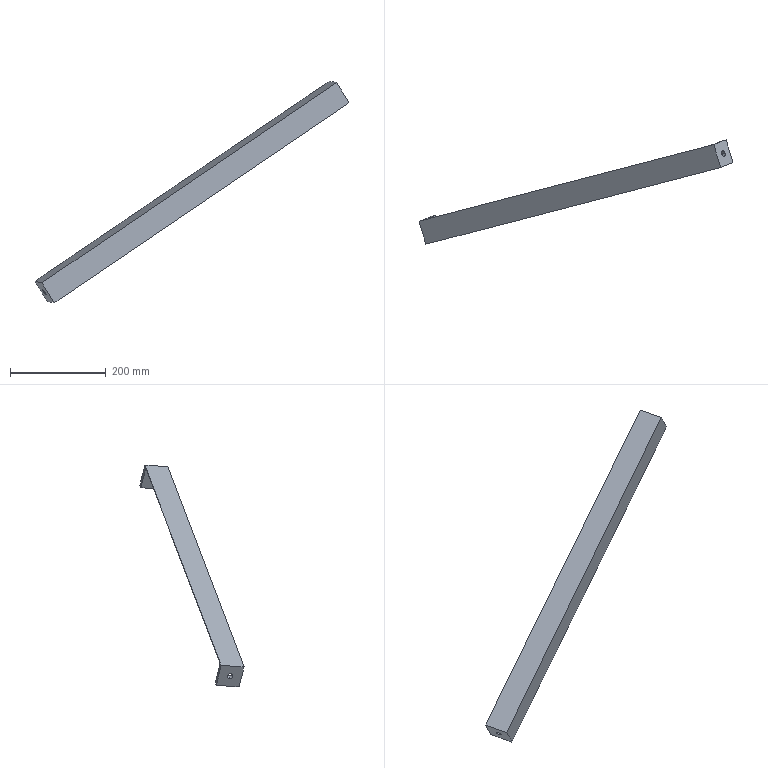Component | SolidWorks | CrusherFrameSpacer-1 | 1 solid | 19 faces | box 654.75 x 217.27 x 462.26 mm | volume 399079 mm3 | plane 12 | cylinder 7 | commonest cylinder face diameters 12 x4 10 x2 14 x1
build123d program:
from build123d import *

# Parameters (mm, degrees)
EXTRUDE2_DEPTH     = 760
SKETCH3_W          = 50
SKETCH3_H          = 50
EXTRUDE3_DEPTH     = 10
SKETCH4_W          = 50
SKETCH4_H          = 50
EXTRUDE4_DEPTH     = 10
SKETCH5_R          = 6
CUT_EXTRUDE1_DEPTH = 763.129


with BuildPart() as part:
    # Sketch2 → Extrude2 (new body)
    with BuildSketch(Plane.XY):
        with BuildLine():
            Line((-22.775, 0), (-22.775, 50))
            ThreePointArc((-22.775, 50), (-19.239, 48.536), (-17.775, 45))
            Line((-17.775, 45), (-17.775, 12))
            ThreePointArc((-17.775, 12), (-15.725, 7.05), (-10.775, 5))
            Line((-10.775, 5), (22.225, 5))
            ThreePointArc((22.225, 5), (25.761, 3.536), (27.225, 0))
            Line((27.225, 0), (-22.775, 0))
        make_face()
    extrude(amount=EXTRUDE2_DEPTH)

    # Sketch3 → Extrude3 (add)
    with BuildSketch(Plane.XY.offset(760)):
        with Locations((2.225, 25)):
            Rectangle(SKETCH3_W, SKETCH3_H)
    extrude(amount=-EXTRUDE3_DEPTH)

    # Sketch4 → Extrude4 (add)
    with BuildSketch(Plane(origin=(0, 0, 0), x_dir=(-1, 0, 0), z_dir=(0, 0, -1))):
        with Locations((-2.225, 25)):
            Rectangle(SKETCH4_W, SKETCH4_H)
    extrude(amount=-EXTRUDE4_DEPTH)

    # Sketch5 → Cut-Extrude1 (cut, through all)
    with BuildSketch(Plane(origin=(0, 0, 0), x_dir=(-1, 0, 0), z_dir=(0, 0, -1))):
        with Locations((-2.225, 25)):
            Circle(SKETCH5_R)
    extrude(amount=-CUT_EXTRUDE1_DEPTH, mode=Mode.SUBTRACT)


solid = part.part

# Placed as in the assembly
solid = solid.moved(Location((-230.699, -92.36, -620.774), (-20.862, 53.982, 29.322)))
STEP:
#1=CARTESIAN_POINT('',(15.001,3.637,-8.21));
#2=VERTEX_POINT('',#1);
#3=CARTESIAN_POINT('',(14.759,3.54,-7.816));
#4=VERTEX_POINT('',#3);
#5=CARTESIAN_POINT('',(14.88,3.589,-8.013));
#6=DIRECTION('',(-0.8088,-0.2094,-0.5495));
#7=DIRECTION('',(-0.5127,-0.2065,0.8334));
#8=AXIS2_PLACEMENT_3D('',#5,#6,#7);
#9=CIRCLE('',#8,0.2362);
#10=EDGE_CURVE('',#2,#4,#9,.T.);
#11=ORIENTED_EDGE('',*,*,#10,.F.);
#12=CARTESIAN_POINT('',(14.683,3.555,-8.426));
#13=VERTEX_POINT('',#12);
#14=CARTESIAN_POINT('',(15.001,3.637,-8.21));
#15=DIRECTION('',(-0.8088,-0.2094,-0.5495));
#16=VECTOR('',#15,39.37);
#17=LINE('',#14,#16);
#18=EDGE_CURVE('',#2,#13,#17,.T.);
#19=ORIENTED_EDGE('',*,*,#18,.T.);
#20=CARTESIAN_POINT('',(14.441,3.457,-8.032));
#21=VERTEX_POINT('',#20);
#22=CARTESIAN_POINT('',(14.562,3.506,-8.229));
#23=DIRECTION('',(0.8088,0.2094,0.5495));
#24=DIRECTION('',(0.5127,0.2065,-0.8334));
#25=AXIS2_PLACEMENT_3D('',#22,#23,#24);
#26=CIRCLE('',#25,0.2362);
#27=EDGE_CURVE('',#21,#13,#26,.T.);
#28=ORIENTED_EDGE('',*,*,#27,.F.);
#29=CARTESIAN_POINT('',(14.759,3.54,-7.816));
#30=DIRECTION('',(-0.8088,-0.2094,-0.5495));
#31=VECTOR('',#30,39.37);
#32=LINE('',#29,#31);
#33=EDGE_CURVE('',#4,#21,#32,.T.);
#34=ORIENTED_EDGE('',*,*,#33,.F.);
#35=EDGE_LOOP('',(#11,#19,#28,#34));
#36=FACE_OUTER_BOUND('',#35,.T.);
#37=CARTESIAN_POINT('',(14.88,3.589,-8.013));
#38=DIRECTION('',(-0.8088,-0.2094,-0.5495));
#39=DIRECTION('',(-0.5127,-0.2065,0.8334));
#40=AXIS2_PLACEMENT_3D('',#37,#38,#39);
#41=CYLINDRICAL_SURFACE('',#40,0.2362);
#42=ADVANCED_FACE('',(#36),#41,.F.);
#43=CARTESIAN_POINT('',(-8.882,-2.546,-24.435));
#44=VERTEX_POINT('',#43);
#45=CARTESIAN_POINT('',(-9.124,-2.644,-24.041));
#46=VERTEX_POINT('',#45);
#47=CARTESIAN_POINT('',(-9.003,-2.595,-24.238));
#48=DIRECTION('',(-0.8088,-0.2094,-0.5495));
#49=DIRECTION('',(-0.5127,-0.2065,0.8334));
#50=AXIS2_PLACEMENT_3D('',#47,#48,#49);
#51=CIRCLE('',#50,0.2362);
#52=EDGE_CURVE('',#44,#46,#51,.T.);
#53=ORIENTED_EDGE('',*,*,#52,.F.);
#54=CARTESIAN_POINT('',(-9.2,-2.629,-24.651));
#55=VERTEX_POINT('',#54);
#56=CARTESIAN_POINT('',(15.001,3.637,-8.21));
#57=DIRECTION('',(-0.8088,-0.2094,-0.5495));
#58=VECTOR('',#57,39.37);
#59=LINE('',#56,#58);
#60=EDGE_CURVE('',#44,#55,#59,.T.);
#61=ORIENTED_EDGE('',*,*,#60,.T.);
#62=CARTESIAN_POINT('',(-9.442,-2.726,-24.257));
#63=VERTEX_POINT('',#62);
#64=CARTESIAN_POINT('',(-9.321,-2.677,-24.454));
#65=DIRECTION('',(-0.8088,-0.2094,-0.5495));
#66=DIRECTION('',(-0.5127,-0.2065,0.8334));
#67=AXIS2_PLACEMENT_3D('',#64,#65,#66);
#68=CIRCLE('',#67,0.2362);
#69=EDGE_CURVE('',#55,#63,#68,.T.);
#70=ORIENTED_EDGE('',*,*,#69,.T.);
#71=CARTESIAN_POINT('',(14.759,3.54,-7.816));
#72=DIRECTION('',(-0.8088,-0.2094,-0.5495));
#73=VECTOR('',#72,39.37);
#74=LINE('',#71,#73);
#75=EDGE_CURVE('',#46,#63,#74,.T.);
#76=ORIENTED_EDGE('',*,*,#75,.F.);
#77=EDGE_LOOP('',(#53,#61,#70,#76));
#78=FACE_OUTER_BOUND('',#77,.T.);
#79=CARTESIAN_POINT('',(14.88,3.589,-8.013));
#80=DIRECTION('',(-0.8088,-0.2094,-0.5495));
#81=DIRECTION('',(-0.5127,-0.2065,0.8334));
#82=AXIS2_PLACEMENT_3D('',#79,#80,#81);
#83=CYLINDRICAL_SURFACE('',#82,0.2362);
#84=ADVANCED_FACE('',(#78),#83,.F.);
#85=CARTESIAN_POINT('',(-8.372,-3.185,-24.941));
#86=VERTEX_POINT('',#85);
#87=CARTESIAN_POINT('',(-8.215,-3.332,-25.117));
#88=VERTEX_POINT('',#87);
#89=CARTESIAN_POINT('',(-8.316,-3.373,-24.953));
#90=DIRECTION('',(-0.8088,-0.2094,-0.5495));
#91=DIRECTION('',(-0.5127,-0.2065,0.8334));
#92=AXIS2_PLACEMENT_3D('',#89,#90,#91);
#93=CIRCLE('',#92,0.1969);
#94=EDGE_CURVE('',#86,#88,#93,.T.);
#95=ORIENTED_EDGE('',*,*,#94,.F.);
#96=CARTESIAN_POINT('',(15.192,2.916,-8.932));
#97=VERTEX_POINT('',#96);
#98=CARTESIAN_POINT('',(15.511,2.999,-8.716));
#99=DIRECTION('',(-0.8088,-0.2094,-0.5495));
#100=VECTOR('',#99,39.37);
#101=LINE('',#98,#100);
#102=EDGE_CURVE('',#97,#86,#101,.T.);
#103=ORIENTED_EDGE('',*,*,#102,.F.);
#104=CARTESIAN_POINT('',(15.35,2.769,-9.108));
#105=VERTEX_POINT('',#104);
#106=CARTESIAN_POINT('',(15.249,2.728,-8.944));
#107=DIRECTION('',(0.8088,0.2094,0.5495));
#108=DIRECTION('',(0.5127,0.2065,-0.8334));
#109=AXIS2_PLACEMENT_3D('',#106,#107,#108);
#110=CIRCLE('',#109,0.1969);
#111=EDGE_CURVE('',#105,#97,#110,.T.);
#112=ORIENTED_EDGE('',*,*,#111,.F.);
#113=CARTESIAN_POINT('',(15.668,2.851,-8.892));
#114=DIRECTION('',(-0.8088,-0.2094,-0.5495));
#115=VECTOR('',#114,39.37);
#116=LINE('',#113,#115);
#117=EDGE_CURVE('',#105,#88,#116,.T.);
#118=ORIENTED_EDGE('',*,*,#117,.T.);
#119=EDGE_LOOP('',(#95,#103,#112,#118));
#120=FACE_OUTER_BOUND('',#119,.T.);
#121=CARTESIAN_POINT('',(15.567,2.81,-8.728));
#122=DIRECTION('',(-0.8088,-0.2094,-0.5495));
#123=DIRECTION('',(-0.5127,-0.2065,0.8334));
#124=AXIS2_PLACEMENT_3D('',#121,#122,#123);
#125=CYLINDRICAL_SURFACE('',#124,0.1969);
#126=ADVANCED_FACE('',(#120),#125,.T.);
#127=CARTESIAN_POINT('',(-9.038,-3.453,-23.858));
#128=VERTEX_POINT('',#127);
#129=CARTESIAN_POINT('',(-8.372,-3.185,-24.941));
#130=DIRECTION('',(0.5127,0.2065,-0.8334));
#131=VECTOR('',#130,39.37);
#132=LINE('',#129,#131);
#133=EDGE_CURVE('',#128,#86,#132,.T.);
#134=ORIENTED_EDGE('',*,*,#133,.F.);
#135=CARTESIAN_POINT('',(14.526,2.648,-7.85));
#136=VERTEX_POINT('',#135);
#137=CARTESIAN_POINT('',(14.845,2.73,-7.633));
#138=DIRECTION('',(-0.8088,-0.2094,-0.5495));
#139=VECTOR('',#138,39.37);
#140=LINE('',#137,#139);
#141=EDGE_CURVE('',#136,#128,#140,.T.);
#142=ORIENTED_EDGE('',*,*,#141,.F.);
#143=CARTESIAN_POINT('',(15.192,2.916,-8.932));
#144=DIRECTION('',(-0.5127,-0.2065,0.8334));
#145=VECTOR('',#144,39.37);
#146=LINE('',#143,#145);
#147=EDGE_CURVE('',#97,#136,#146,.T.);
#148=ORIENTED_EDGE('',*,*,#147,.F.);
#149=ORIENTED_EDGE('',*,*,#102,.T.);
#150=EDGE_LOOP('',(#134,#142,#148,#149));
#151=FACE_OUTER_BOUND('',#150,.T.);
#152=CARTESIAN_POINT('',(15.511,2.999,-8.716));
#153=DIRECTION('',(0.288,-0.9558,-0.05964));
#154=DIRECTION('',(0.5127,0.2065,-0.8334));
#155=AXIS2_PLACEMENT_3D('',#152,#153,#154);
#156=PLANE('',#155);
#157=ADVANCED_FACE('',(#151),#156,.F.);
#158=CARTESIAN_POINT('',(-9.259,-3.247,-23.612));
#159=VERTEX_POINT('',#158);
#160=CARTESIAN_POINT('',(-9.118,-3.19,-23.842));
#161=DIRECTION('',(0.8088,0.2094,0.5495));
#162=DIRECTION('',(-0.5127,-0.2065,0.8334));
#163=AXIS2_PLACEMENT_3D('',#160,#161,#162);
#164=CIRCLE('',#163,0.2756);
#165=EDGE_CURVE('',#159,#128,#164,.T.);
#166=ORIENTED_EDGE('',*,*,#165,.F.);
#167=CARTESIAN_POINT('',(14.305,2.854,-7.604));
#168=VERTEX_POINT('',#167);
#169=CARTESIAN_POINT('',(14.624,2.937,-7.387));
#170=DIRECTION('',(-0.8088,-0.2094,-0.5495));
#171=VECTOR('',#170,39.37);
#172=LINE('',#169,#171);
#173=EDGE_CURVE('',#168,#159,#172,.T.);
#174=ORIENTED_EDGE('',*,*,#173,.F.);
#175=CARTESIAN_POINT('',(14.447,2.911,-7.833));
#176=DIRECTION('',(-0.8088,-0.2094,-0.5495));
#177=DIRECTION('',(0.5127,0.2065,-0.8334));
#178=AXIS2_PLACEMENT_3D('',#175,#176,#177);
#179=CIRCLE('',#178,0.2756);
#180=EDGE_CURVE('',#136,#168,#179,.T.);
#181=ORIENTED_EDGE('',*,*,#180,.F.);
#182=ORIENTED_EDGE('',*,*,#141,.T.);
#183=EDGE_LOOP('',(#166,#174,#181,#182));
#184=FACE_OUTER_BOUND('',#183,.T.);
#185=CARTESIAN_POINT('',(14.765,2.994,-7.617));
#186=DIRECTION('',(-0.8088,-0.2094,-0.5495));
#187=DIRECTION('',(-0.5127,-0.2065,0.8334));
#188=AXIS2_PLACEMENT_3D('',#185,#186,#187);
#189=CYLINDRICAL_SURFACE('',#188,0.2756);
#190=ADVANCED_FACE('',(#184),#189,.F.);
#191=CARTESIAN_POINT('',(-9.633,-2.005,-23.535));
#192=VERTEX_POINT('',#191);
#193=CARTESIAN_POINT('',(-9.633,-2.005,-23.535));
#194=DIRECTION('',(0.288,-0.9558,-0.05964));
#195=VECTOR('',#194,39.37);
#196=LINE('',#193,#195);
#197=EDGE_CURVE('',#192,#159,#196,.T.);
#198=ORIENTED_EDGE('',*,*,#197,.F.);
#199=CARTESIAN_POINT('',(13.931,4.096,-7.526));
#200=VERTEX_POINT('',#199);
#201=CARTESIAN_POINT('',(14.25,4.179,-7.31));
#202=DIRECTION('',(-0.8088,-0.2094,-0.5495));
#203=VECTOR('',#202,39.37);
#204=LINE('',#201,#203);
#205=EDGE_CURVE('',#200,#192,#204,.T.);
#206=ORIENTED_EDGE('',*,*,#205,.F.);
#207=CARTESIAN_POINT('',(13.931,4.096,-7.526));
#208=DIRECTION('',(-0.288,0.9558,0.05964));
#209=VECTOR('',#208,39.37);
#210=LINE('',#207,#209);
#211=EDGE_CURVE('',#168,#200,#210,.T.);
#212=ORIENTED_EDGE('',*,*,#211,.F.);
#213=ORIENTED_EDGE('',*,*,#173,.T.);
#214=EDGE_LOOP('',(#198,#206,#212,#213));
#215=FACE_OUTER_BOUND('',#214,.T.);
#216=CARTESIAN_POINT('',(14.25,4.179,-7.31));
#217=DIRECTION('',(-0.5127,-0.2065,0.8334));
#218=DIRECTION('',(0.288,-0.9558,-0.05964));
#219=AXIS2_PLACEMENT_3D('',#216,#217,#218);
#220=PLANE('',#219);
#221=ADVANCED_FACE('',(#215),#220,.F.);
#222=CARTESIAN_POINT('',(-9.791,-1.857,-23.359));
#223=VERTEX_POINT('',#222);
#224=CARTESIAN_POINT('',(-9.734,-2.046,-23.371));
#225=DIRECTION('',(-0.8088,-0.2094,-0.5495));
#226=DIRECTION('',(-0.5127,-0.2065,0.8334));
#227=AXIS2_PLACEMENT_3D('',#224,#225,#226);
#228=CIRCLE('',#227,0.1969);
#229=EDGE_CURVE('',#223,#192,#228,.T.);
#230=ORIENTED_EDGE('',*,*,#229,.F.);
#231=CARTESIAN_POINT('',(13.774,4.244,-7.35));
#232=VERTEX_POINT('',#231);
#233=CARTESIAN_POINT('',(14.092,4.326,-7.134));
#234=DIRECTION('',(-0.8088,-0.2094,-0.5495));
#235=VECTOR('',#234,39.37);
#236=LINE('',#233,#235);
#237=EDGE_CURVE('',#232,#223,#236,.T.);
#238=ORIENTED_EDGE('',*,*,#237,.F.);
#239=CARTESIAN_POINT('',(13.83,4.055,-7.362));
#240=DIRECTION('',(0.8088,0.2094,0.5495));
#241=DIRECTION('',(0.5127,0.2065,-0.8334));
#242=AXIS2_PLACEMENT_3D('',#239,#240,#241);
#243=CIRCLE('',#242,0.1969);
#244=EDGE_CURVE('',#200,#232,#243,.T.);
#245=ORIENTED_EDGE('',*,*,#244,.F.);
#246=ORIENTED_EDGE('',*,*,#205,.T.);
#247=EDGE_LOOP('',(#230,#238,#245,#246));
#248=FACE_OUTER_BOUND('',#247,.T.);
#249=CARTESIAN_POINT('',(14.149,4.138,-7.146));
#250=DIRECTION('',(-0.8088,-0.2094,-0.5495));
#251=DIRECTION('',(-0.5127,-0.2065,0.8334));
#252=AXIS2_PLACEMENT_3D('',#249,#250,#251);
#253=CYLINDRICAL_SURFACE('',#252,0.1969);
#254=ADVANCED_FACE('',(#248),#253,.T.);
#255=CARTESIAN_POINT('',(-8.533,-3.415,-25.333));
#256=VERTEX_POINT('',#255);
#257=CARTESIAN_POINT('',(-8.215,-3.332,-25.117));
#258=DIRECTION('',(-0.8088,-0.2094,-0.5495));
#259=VECTOR('',#258,39.37);
#260=LINE('',#257,#259);
#261=EDGE_CURVE('',#88,#256,#260,.T.);
#262=ORIENTED_EDGE('',*,*,#261,.F.);
#263=ORIENTED_EDGE('',*,*,#117,.F.);
#264=CARTESIAN_POINT('',(15.668,2.851,-8.892));
#265=VERTEX_POINT('',#264);
#266=CARTESIAN_POINT('',(15.668,2.851,-8.892));
#267=DIRECTION('',(-0.8088,-0.2094,-0.5495));
#268=VECTOR('',#267,39.37);
#269=LINE('',#266,#268);
#270=EDGE_CURVE('',#265,#105,#269,.T.);
#271=ORIENTED_EDGE('',*,*,#270,.F.);
#272=CARTESIAN_POINT('',(14.659,2.445,-7.251));
#273=VERTEX_POINT('',#272);
#274=CARTESIAN_POINT('',(14.659,2.445,-7.251));
#275=DIRECTION('',(0.5127,0.2065,-0.8334));
#276=VECTOR('',#275,39.37);
#277=LINE('',#274,#276);
#278=EDGE_CURVE('',#273,#265,#277,.T.);
#279=ORIENTED_EDGE('',*,*,#278,.F.);
#280=CARTESIAN_POINT('',(-9.542,-3.821,-23.693));
#281=VERTEX_POINT('',#280);
#282=CARTESIAN_POINT('',(14.659,2.445,-7.251));
#283=DIRECTION('',(-0.8088,-0.2094,-0.5495));
#284=VECTOR('',#283,39.37);
#285=LINE('',#282,#284);
#286=EDGE_CURVE('',#273,#281,#285,.T.);
#287=ORIENTED_EDGE('',*,*,#286,.T.);
#288=CARTESIAN_POINT('',(-9.542,-3.821,-23.693));
#289=DIRECTION('',(0.5127,0.2065,-0.8334));
#290=VECTOR('',#289,39.37);
#291=LINE('',#288,#290);
#292=EDGE_CURVE('',#281,#256,#291,.T.);
#293=ORIENTED_EDGE('',*,*,#292,.T.);
#294=EDGE_LOOP('',(#262,#263,#271,#279,#287,#293));
#295=FACE_OUTER_BOUND('',#294,.T.);
#296=CARTESIAN_POINT('',(14.659,2.445,-7.251));
#297=DIRECTION('',(-0.288,0.9558,0.05964));
#298=DIRECTION('',(-0.5127,-0.2065,0.8334));
#299=AXIS2_PLACEMENT_3D('',#296,#297,#298);
#300=PLANE('',#299);
#301=ADVANCED_FACE('',(#295),#300,.F.);
#302=CARTESIAN_POINT('',(-10.109,-1.94,-23.575));
#303=VERTEX_POINT('',#302);
#304=CARTESIAN_POINT('',(-9.542,-3.821,-23.693));
#305=DIRECTION('',(0.288,-0.9558,-0.05964));
#306=VECTOR('',#305,39.37);
#307=LINE('',#304,#306);
#308=EDGE_CURVE('',#303,#281,#307,.T.);
#309=ORIENTED_EDGE('',*,*,#308,.T.);
#310=ORIENTED_EDGE('',*,*,#286,.F.);
#311=CARTESIAN_POINT('',(14.092,4.326,-7.134));
#312=VERTEX_POINT('',#311);
#313=CARTESIAN_POINT('',(14.659,2.445,-7.251));
#314=DIRECTION('',(0.288,-0.9558,-0.05964));
#315=VECTOR('',#314,39.37);
#316=LINE('',#313,#315);
#317=EDGE_CURVE('',#312,#273,#316,.T.);
#318=ORIENTED_EDGE('',*,*,#317,.F.);
#319=CARTESIAN_POINT('',(14.092,4.326,-7.134));
#320=DIRECTION('',(-0.8088,-0.2094,-0.5495));
#321=VECTOR('',#320,39.37);
#322=LINE('',#319,#321);
#323=EDGE_CURVE('',#312,#232,#322,.T.);
#324=ORIENTED_EDGE('',*,*,#323,.T.);
#325=ORIENTED_EDGE('',*,*,#237,.T.);
#326=CARTESIAN_POINT('',(-9.791,-1.857,-23.359));
#327=DIRECTION('',(-0.8088,-0.2094,-0.5495));
#328=VECTOR('',#327,39.37);
#329=LINE('',#326,#328);
#330=EDGE_CURVE('',#223,#303,#329,.T.);
#331=ORIENTED_EDGE('',*,*,#330,.T.);
#332=EDGE_LOOP('',(#309,#310,#318,#324,#325,#331));
#333=FACE_OUTER_BOUND('',#332,.T.);
#334=CARTESIAN_POINT('',(14.659,2.445,-7.251));
#335=DIRECTION('',(0.5127,0.2065,-0.8334));
#336=DIRECTION('',(-0.288,0.9558,0.05964));
#337=AXIS2_PLACEMENT_3D('',#334,#335,#336);
#338=PLANE('',#337);
#339=ADVANCED_FACE('',(#333),#338,.F.);
#340=CARTESIAN_POINT('',(14.88,3.589,-8.013));
#341=DIRECTION('',(-0.8088,-0.2094,-0.5495));
#342=DIRECTION('',(-0.5127,-0.2065,0.8334));
#343=AXIS2_PLACEMENT_3D('',#340,#341,#342);
#344=CIRCLE('',#343,0.2362);
#345=EDGE_CURVE('',#4,#2,#344,.T.);
#346=ORIENTED_EDGE('',*,*,#345,.T.);
#347=ORIENTED_EDGE('',*,*,#10,.T.);
#348=EDGE_LOOP('',(#346,#347));
#349=FACE_BOUND('',#348,.T.);
#350=ORIENTED_EDGE('',*,*,#278,.T.);
#351=CARTESIAN_POINT('',(15.101,4.733,-8.775));
#352=VERTEX_POINT('',#351);
#353=CARTESIAN_POINT('',(15.668,2.851,-8.892));
#354=DIRECTION('',(-0.288,0.9558,0.05964));
#355=VECTOR('',#354,39.37);
#356=LINE('',#353,#355);
#357=EDGE_CURVE('',#265,#352,#356,.T.);
#358=ORIENTED_EDGE('',*,*,#357,.T.);
#359=CARTESIAN_POINT('',(15.101,4.733,-8.775));
#360=DIRECTION('',(-0.5127,-0.2065,0.8334));
#361=VECTOR('',#360,39.37);
#362=LINE('',#359,#361);
#363=EDGE_CURVE('',#352,#312,#362,.T.);
#364=ORIENTED_EDGE('',*,*,#363,.T.);
#365=ORIENTED_EDGE('',*,*,#317,.T.);
#366=EDGE_LOOP('',(#350,#358,#364,#365));
#367=FACE_OUTER_BOUND('',#366,.T.);
#368=CARTESIAN_POINT('',(15.567,2.81,-8.728));
#369=DIRECTION('',(-0.8088,-0.2094,-0.5495));
#370=DIRECTION('',(-0.5127,-0.2065,0.8334));
#371=AXIS2_PLACEMENT_3D('',#368,#369,#370);
#372=PLANE('',#371);
#373=ADVANCED_FACE('',(#349,#367),#372,.F.);
#374=CARTESIAN_POINT('',(-9.321,-2.677,-24.454));
#375=DIRECTION('',(-0.8088,-0.2094,-0.5495));
#376=DIRECTION('',(-0.5127,-0.2065,0.8334));
#377=AXIS2_PLACEMENT_3D('',#374,#375,#376);
#378=CIRCLE('',#377,0.2362);
#379=EDGE_CURVE('',#63,#55,#378,.T.);
#380=ORIENTED_EDGE('',*,*,#379,.F.);
#381=ORIENTED_EDGE('',*,*,#69,.F.);
#382=EDGE_LOOP('',(#380,#381));
#383=FACE_BOUND('',#382,.T.);
#384=ORIENTED_EDGE('',*,*,#292,.F.);
#385=ORIENTED_EDGE('',*,*,#308,.F.);
#386=CARTESIAN_POINT('',(-9.1,-1.533,-25.216));
#387=VERTEX_POINT('',#386);
#388=CARTESIAN_POINT('',(-9.1,-1.533,-25.216));
#389=DIRECTION('',(0.5127,0.2065,-0.8334));
#390=VECTOR('',#389,39.37);
#391=LINE('',#388,#390);
#392=EDGE_CURVE('',#303,#387,#391,.T.);
#393=ORIENTED_EDGE('',*,*,#392,.T.);
#394=CARTESIAN_POINT('',(-9.1,-1.533,-25.216));
#395=DIRECTION('',(0.288,-0.9558,-0.05964));
#396=VECTOR('',#395,39.37);
#397=LINE('',#394,#396);
#398=EDGE_CURVE('',#387,#256,#397,.T.);
#399=ORIENTED_EDGE('',*,*,#398,.T.);
#400=EDGE_LOOP('',(#384,#385,#393,#399));
#401=FACE_OUTER_BOUND('',#400,.T.);
#402=CARTESIAN_POINT('',(-8.634,-3.456,-25.169));
#403=DIRECTION('',(-0.8088,-0.2094,-0.5495));
#404=DIRECTION('',(-0.5127,-0.2065,0.8334));
#405=AXIS2_PLACEMENT_3D('',#402,#403,#404);
#406=PLANE('',#405);
#407=ADVANCED_FACE('',(#383,#401),#406,.T.);
#408=ORIENTED_EDGE('',*,*,#27,.T.);
#409=CARTESIAN_POINT('',(14.562,3.506,-8.229));
#410=DIRECTION('',(0.8088,0.2094,0.5495));
#411=DIRECTION('',(0.5127,0.2065,-0.8334));
#412=AXIS2_PLACEMENT_3D('',#409,#410,#411);
#413=CIRCLE('',#412,0.2362);
#414=EDGE_CURVE('',#13,#21,#413,.T.);
#415=ORIENTED_EDGE('',*,*,#414,.T.);
#416=EDGE_LOOP('',(#408,#415));
#417=FACE_BOUND('',#416,.T.);
#418=CARTESIAN_POINT('',(14.783,4.65,-8.991));
#419=VERTEX_POINT('',#418);
#420=CARTESIAN_POINT('',(15.35,2.769,-9.108));
#421=DIRECTION('',(-0.288,0.9558,0.05964));
#422=VECTOR('',#421,39.37);
#423=LINE('',#420,#422);
#424=EDGE_CURVE('',#105,#419,#423,.T.);
#425=ORIENTED_EDGE('',*,*,#424,.F.);
#426=ORIENTED_EDGE('',*,*,#111,.T.);
#427=ORIENTED_EDGE('',*,*,#147,.T.);
#428=ORIENTED_EDGE('',*,*,#180,.T.);
#429=ORIENTED_EDGE('',*,*,#211,.T.);
#430=ORIENTED_EDGE('',*,*,#244,.T.);
#431=CARTESIAN_POINT('',(14.783,4.65,-8.991));
#432=DIRECTION('',(-0.5127,-0.2065,0.8334));
#433=VECTOR('',#432,39.37);
#434=LINE('',#431,#433);
#435=EDGE_CURVE('',#419,#232,#434,.T.);
#436=ORIENTED_EDGE('',*,*,#435,.F.);
#437=EDGE_LOOP('',(#425,#426,#427,#428,#429,#430,#436));
#438=FACE_OUTER_BOUND('',#437,.T.);
#439=CARTESIAN_POINT('',(14.783,4.65,-8.991));
#440=DIRECTION('',(0.8088,0.2094,0.5495));
#441=DIRECTION('',(0.5127,0.2065,-0.8334));
#442=AXIS2_PLACEMENT_3D('',#439,#440,#441);
#443=PLANE('',#442);
#444=ADVANCED_FACE('',(#417,#438),#443,.F.);
#445=ORIENTED_EDGE('',*,*,#357,.F.);
#446=ORIENTED_EDGE('',*,*,#270,.T.);
#447=ORIENTED_EDGE('',*,*,#424,.T.);
#448=CARTESIAN_POINT('',(14.783,4.65,-8.991));
#449=DIRECTION('',(0.8088,0.2094,0.5495));
#450=VECTOR('',#449,39.37);
#451=LINE('',#448,#450);
#452=EDGE_CURVE('',#419,#352,#451,.T.);
#453=ORIENTED_EDGE('',*,*,#452,.T.);
#454=EDGE_LOOP('',(#445,#446,#447,#453));
#455=FACE_OUTER_BOUND('',#454,.T.);
#456=CARTESIAN_POINT('',(15.35,2.769,-9.108));
#457=DIRECTION('',(0.5127,0.2065,-0.8334));
#458=DIRECTION('',(-0.8088,-0.2094,-0.5495));
#459=AXIS2_PLACEMENT_3D('',#456,#457,#458);
#460=PLANE('',#459);
#461=ADVANCED_FACE('',(#455),#460,.T.);
#462=ORIENTED_EDGE('',*,*,#363,.F.);
#463=ORIENTED_EDGE('',*,*,#452,.F.);
#464=ORIENTED_EDGE('',*,*,#435,.T.);
#465=ORIENTED_EDGE('',*,*,#323,.F.);
#466=EDGE_LOOP('',(#462,#463,#464,#465));
#467=FACE_OUTER_BOUND('',#466,.T.);
#468=CARTESIAN_POINT('',(14.783,4.65,-8.991));
#469=DIRECTION('',(-0.288,0.9558,0.05964));
#470=DIRECTION('',(0.8088,0.2094,0.5495));
#471=AXIS2_PLACEMENT_3D('',#468,#469,#470);
#472=PLANE('',#471);
#473=ADVANCED_FACE('',(#467),#472,.T.);
#474=CARTESIAN_POINT('',(-9.003,-2.595,-24.238));
#475=DIRECTION('',(-0.8088,-0.2094,-0.5495));
#476=DIRECTION('',(-0.5127,-0.2065,0.8334));
#477=AXIS2_PLACEMENT_3D('',#474,#475,#476);
#478=CIRCLE('',#477,0.2362);
#479=EDGE_CURVE('',#46,#44,#478,.T.);
#480=ORIENTED_EDGE('',*,*,#479,.T.);
#481=ORIENTED_EDGE('',*,*,#52,.T.);
#482=EDGE_LOOP('',(#480,#481));
#483=FACE_BOUND('',#482,.T.);
#484=ORIENTED_EDGE('',*,*,#133,.T.);
#485=ORIENTED_EDGE('',*,*,#94,.T.);
#486=CARTESIAN_POINT('',(-8.782,-1.451,-24.999));
#487=VERTEX_POINT('',#486);
#488=CARTESIAN_POINT('',(-8.782,-1.451,-24.999));
#489=DIRECTION('',(0.288,-0.9558,-0.05964));
#490=VECTOR('',#489,39.37);
#491=LINE('',#488,#490);
#492=EDGE_CURVE('',#487,#88,#491,.T.);
#493=ORIENTED_EDGE('',*,*,#492,.F.);
#494=CARTESIAN_POINT('',(-8.782,-1.451,-24.999));
#495=DIRECTION('',(0.5127,0.2065,-0.8334));
#496=VECTOR('',#495,39.37);
#497=LINE('',#494,#496);
#498=EDGE_CURVE('',#223,#487,#497,.T.);
#499=ORIENTED_EDGE('',*,*,#498,.F.);
#500=ORIENTED_EDGE('',*,*,#229,.T.);
#501=ORIENTED_EDGE('',*,*,#197,.T.);
#502=ORIENTED_EDGE('',*,*,#165,.T.);
#503=EDGE_LOOP('',(#484,#485,#493,#499,#500,#501,#502));
#504=FACE_OUTER_BOUND('',#503,.T.);
#505=CARTESIAN_POINT('',(-8.215,-3.332,-25.117));
#506=DIRECTION('',(-0.8088,-0.2094,-0.5495));
#507=DIRECTION('',(-0.5127,-0.2065,0.8334));
#508=AXIS2_PLACEMENT_3D('',#505,#506,#507);
#509=PLANE('',#508);
#510=ADVANCED_FACE('',(#483,#504),#509,.F.);
#511=ORIENTED_EDGE('',*,*,#398,.F.);
#512=CARTESIAN_POINT('',(-8.782,-1.451,-24.999));
#513=DIRECTION('',(-0.8088,-0.2094,-0.5495));
#514=VECTOR('',#513,39.37);
#515=LINE('',#512,#514);
#516=EDGE_CURVE('',#487,#387,#515,.T.);
#517=ORIENTED_EDGE('',*,*,#516,.F.);
#518=ORIENTED_EDGE('',*,*,#492,.T.);
#519=ORIENTED_EDGE('',*,*,#261,.T.);
#520=EDGE_LOOP('',(#511,#517,#518,#519));
#521=FACE_OUTER_BOUND('',#520,.T.);
#522=CARTESIAN_POINT('',(-8.782,-1.451,-24.999));
#523=DIRECTION('',(0.5127,0.2065,-0.8334));
#524=DIRECTION('',(-0.8088,-0.2094,-0.5495));
#525=AXIS2_PLACEMENT_3D('',#522,#523,#524);
#526=PLANE('',#525);
#527=ADVANCED_FACE('',(#521),#526,.T.);
#528=ORIENTED_EDGE('',*,*,#392,.F.);
#529=ORIENTED_EDGE('',*,*,#330,.F.);
#530=ORIENTED_EDGE('',*,*,#498,.T.);
#531=ORIENTED_EDGE('',*,*,#516,.T.);
#532=EDGE_LOOP('',(#528,#529,#530,#531));
#533=FACE_OUTER_BOUND('',#532,.T.);
#534=CARTESIAN_POINT('',(-8.782,-1.451,-24.999));
#535=DIRECTION('',(-0.288,0.9558,0.05964));
#536=DIRECTION('',(0.8088,0.2094,0.5495));
#537=AXIS2_PLACEMENT_3D('',#534,#535,#536);
#538=PLANE('',#537);
#539=ADVANCED_FACE('',(#533),#538,.T.);
#540=ORIENTED_EDGE('',*,*,#60,.F.);
#541=ORIENTED_EDGE('',*,*,#479,.F.);
#542=ORIENTED_EDGE('',*,*,#75,.T.);
#543=ORIENTED_EDGE('',*,*,#379,.T.);
#544=EDGE_LOOP('',(#540,#541,#542,#543));
#545=FACE_OUTER_BOUND('',#544,.T.);
#546=CARTESIAN_POINT('',(14.88,3.589,-8.013));
#547=DIRECTION('',(-0.8088,-0.2094,-0.5495));
#548=DIRECTION('',(-0.5127,-0.2065,0.8334));
#549=AXIS2_PLACEMENT_3D('',#546,#547,#548);
#550=CYLINDRICAL_SURFACE('',#549,0.2362);
#551=ADVANCED_FACE('',(#545),#550,.F.);
#552=ORIENTED_EDGE('',*,*,#18,.F.);
#553=ORIENTED_EDGE('',*,*,#345,.F.);
#554=ORIENTED_EDGE('',*,*,#33,.T.);
#555=ORIENTED_EDGE('',*,*,#414,.F.);
#556=EDGE_LOOP('',(#552,#553,#554,#555));
#557=FACE_OUTER_BOUND('',#556,.T.);
#558=CARTESIAN_POINT('',(14.88,3.589,-8.013));
#559=DIRECTION('',(-0.8088,-0.2094,-0.5495));
#560=DIRECTION('',(-0.5127,-0.2065,0.8334));
#561=AXIS2_PLACEMENT_3D('',#558,#559,#560);
#562=CYLINDRICAL_SURFACE('',#561,0.2362);
#563=ADVANCED_FACE('',(#557),#562,.F.);
#564=CLOSED_SHELL('',(#42,#84,#126,#157,#190,#221,#254,#301,#339,#373,#407,#444,#461,#473,#510,#527,#539,#551,#563));
#565=MANIFOLD_SOLID_BREP('',#564);
#566=CARTESIAN_POINT('',(0.,0.,0.));
#567=DIRECTION('',(0.,0.,1.));
#568=DIRECTION('',(1.,0.,0.));
#569=AXIS2_PLACEMENT_3D('',#566,#567,#568);
#570=(LENGTH_UNIT()NAMED_UNIT(*)SI_UNIT($,.METRE.));
#571=LENGTH_MEASURE_WITH_UNIT(LENGTH_MEASURE(0.0254),#570);
#572=DIMENSIONAL_EXPONENTS(1.,0.,0.,0.,0.,0.,0.);
#573=(CONVERSION_BASED_UNIT('',#571)LENGTH_UNIT()NAMED_UNIT(#572));
#574=UNCERTAINTY_MEASURE_WITH_UNIT(LENGTH_MEASURE(0.00001),#573,'','');
#575=(NAMED_UNIT(*)PLANE_ANGLE_UNIT()SI_UNIT($,.RADIAN.));
#576=(NAMED_UNIT(*)SI_UNIT($,.STERADIAN.)SOLID_ANGLE_UNIT());
#577=(GEOMETRIC_REPRESENTATION_CONTEXT(3)GLOBAL_UNCERTAINTY_ASSIGNED_CONTEXT((#574))GLOBAL_UNIT_ASSIGNED_CONTEXT((#573,#575,#576))REPRESENTATION_CONTEXT('',''));
#578=ADVANCED_BREP_SHAPE_REPRESENTATION('',(#565,#569),#577);
#579=COLOUR_RGB('',0.7922,0.8196,0.9333);
#580=FILL_AREA_STYLE_COLOUR('',#579);
#581=FILL_AREA_STYLE('',(#580));
#582=SURFACE_STYLE_FILL_AREA(#581);
#583=SURFACE_SIDE_STYLE('',(#582));
#584=SURFACE_STYLE_USAGE(.BOTH.,#583);
#585=PRESENTATION_STYLE_ASSIGNMENT((#584));
#586=STYLED_ITEM('',(#585),#565);
#587=(LENGTH_UNIT()NAMED_UNIT(*)SI_UNIT($,.METRE.));
#588=LENGTH_MEASURE_WITH_UNIT(LENGTH_MEASURE(0.0254),#587);
#589=DIMENSIONAL_EXPONENTS(1.,0.,0.,0.,0.,0.,0.);
#590=(CONVERSION_BASED_UNIT('',#588)LENGTH_UNIT()NAMED_UNIT(#589));
#591=UNCERTAINTY_MEASURE_WITH_UNIT(LENGTH_MEASURE(0.00001),#590,'','');
#592=(NAMED_UNIT(*)PLANE_ANGLE_UNIT()SI_UNIT($,.RADIAN.));
#593=(NAMED_UNIT(*)SI_UNIT($,.STERADIAN.)SOLID_ANGLE_UNIT());
#594=(GEOMETRIC_REPRESENTATION_CONTEXT(3)GLOBAL_UNCERTAINTY_ASSIGNED_CONTEXT((#591))GLOBAL_UNIT_ASSIGNED_CONTEXT((#590,#592,#593))REPRESENTATION_CONTEXT('',''));
#595=MECHANICAL_DESIGN_GEOMETRIC_PRESENTATION_REPRESENTATION('',(#586),#594);
#596=PRESENTATION_LAYER_ASSIGNMENT('','',(#586));